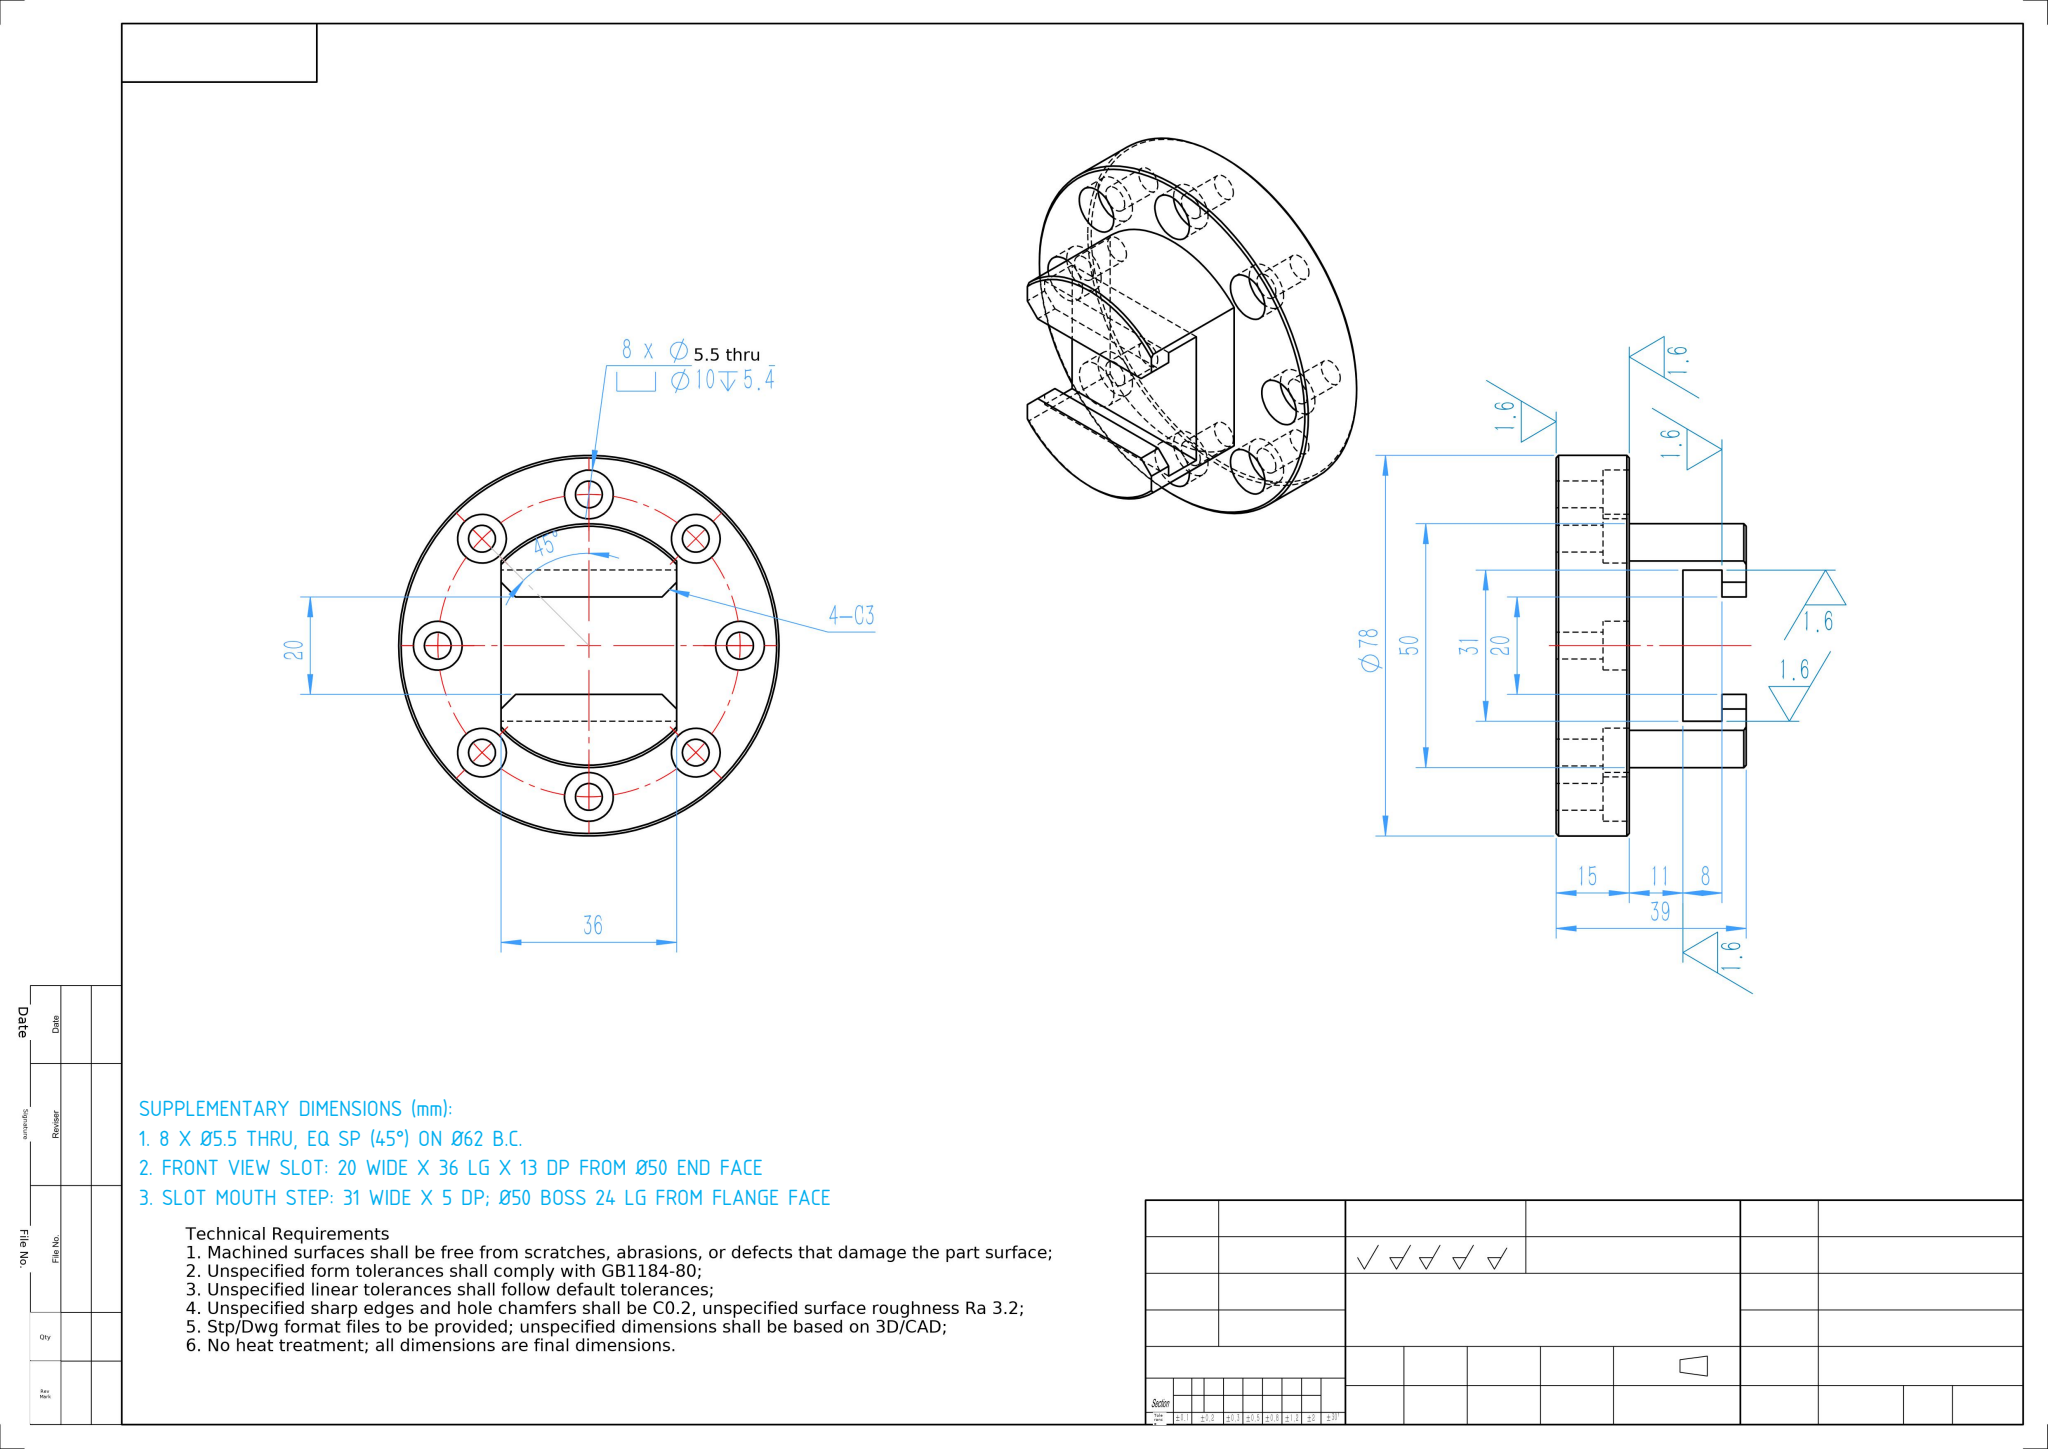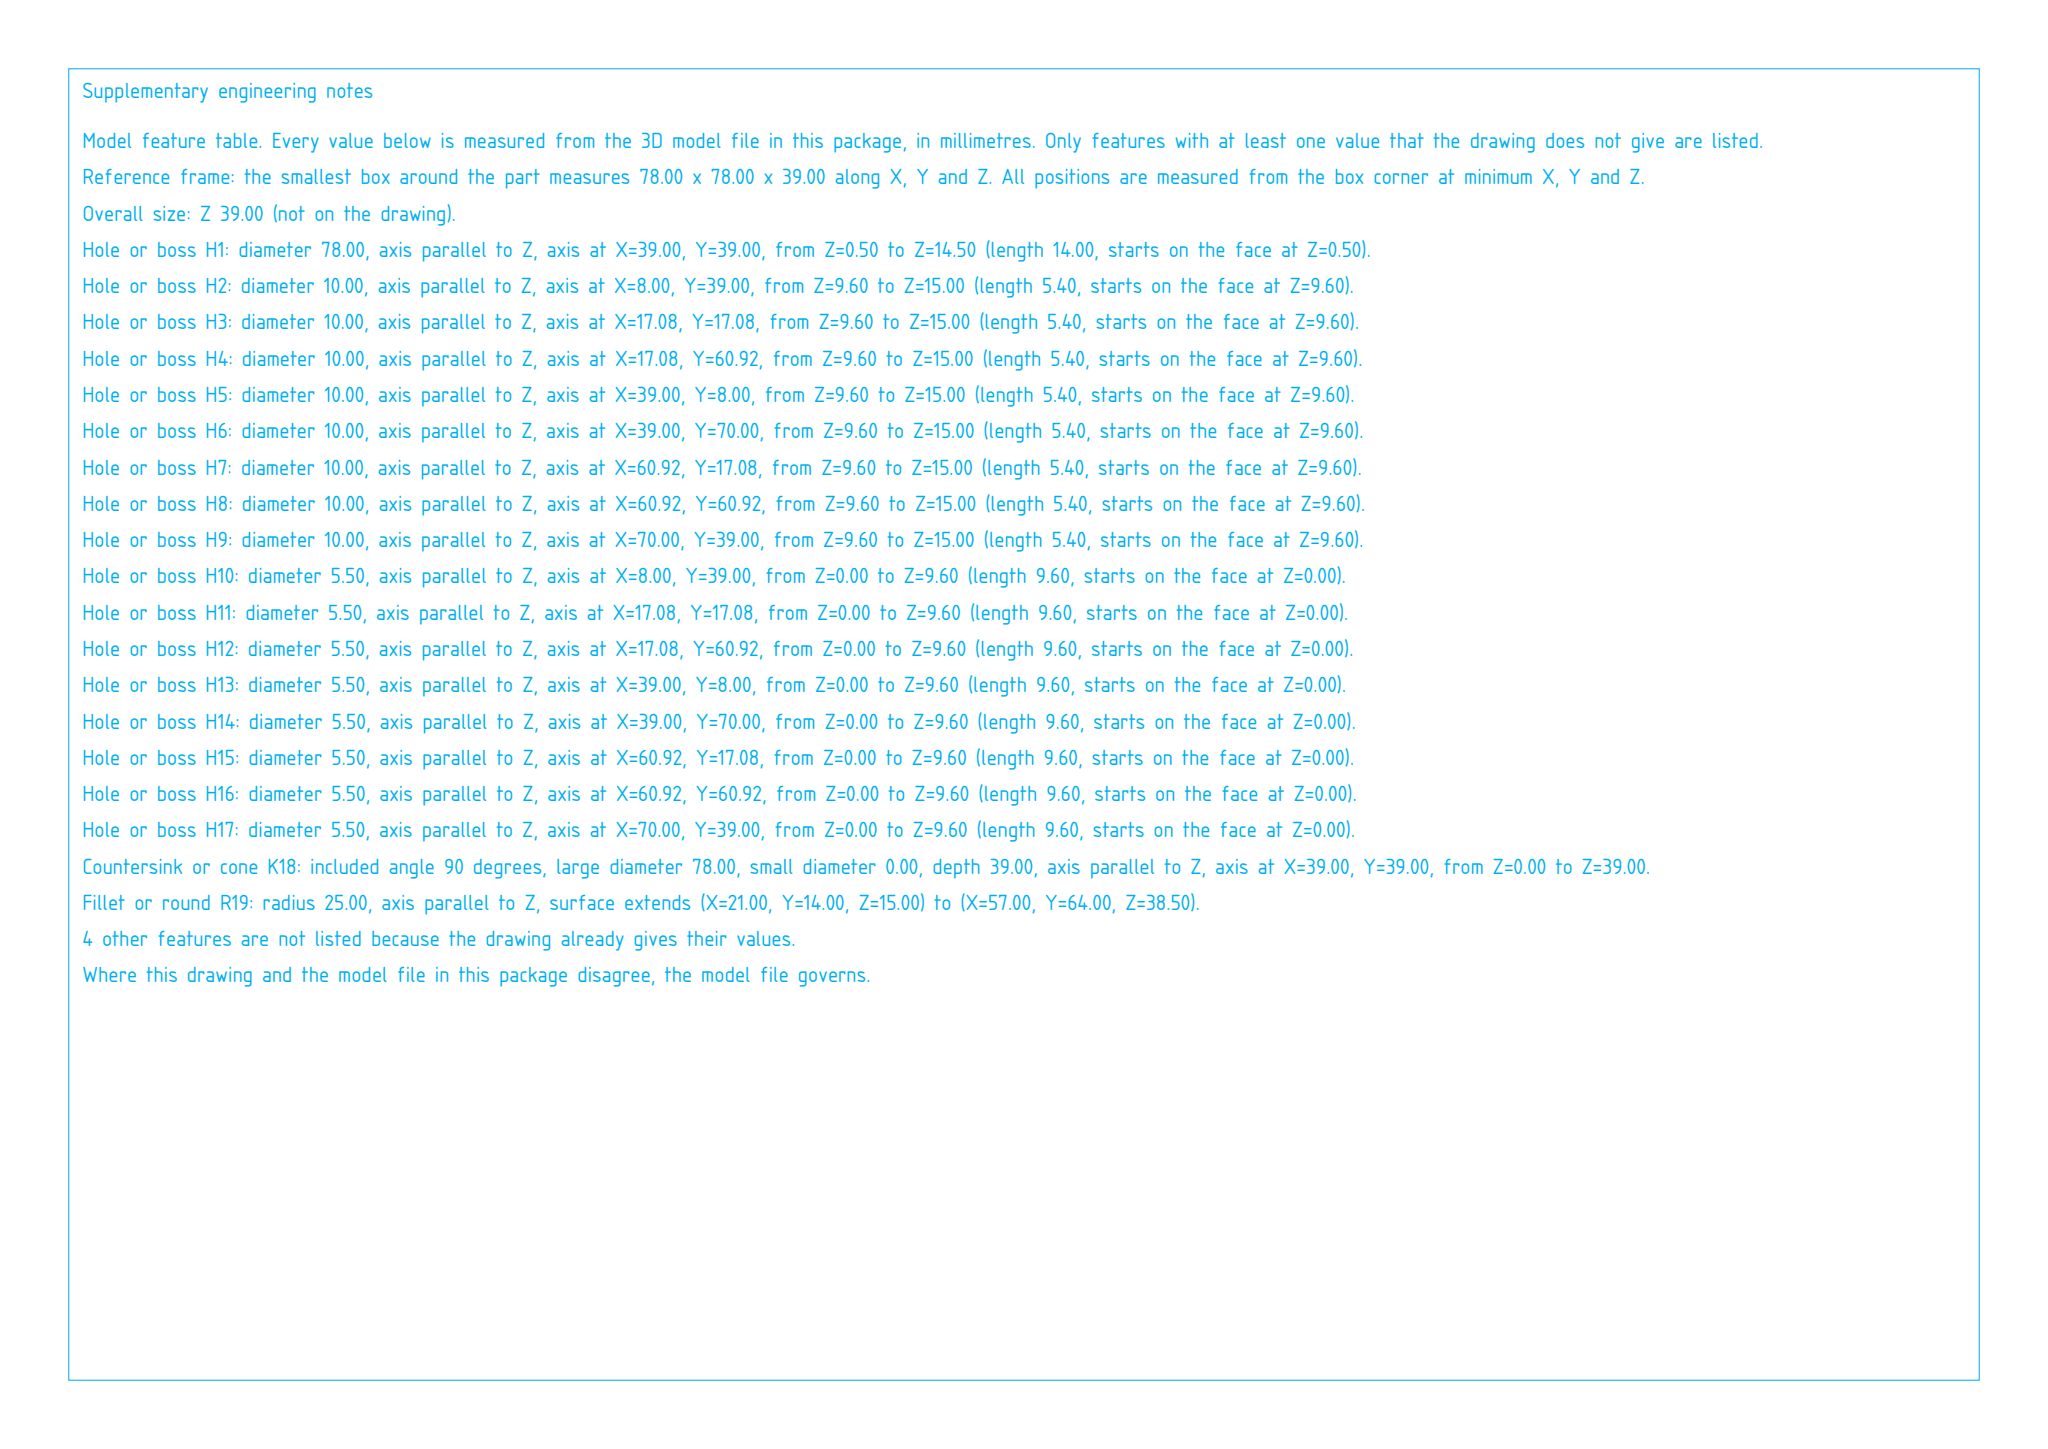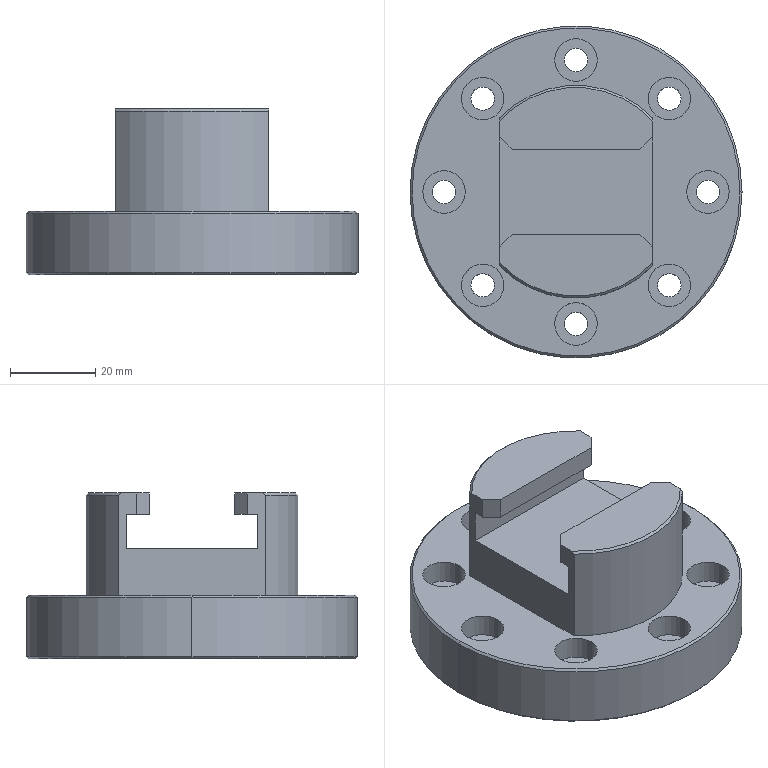Part | SolidWorks | mm | 1 solid | 67 faces | box 78 x 78 x 39 mm | volume 92873 mm3 | cylinder 36 | plane 25 | cone 6 | commonest cylinder face diameters 10 x16 5.5 x16 78 x2 50 x2